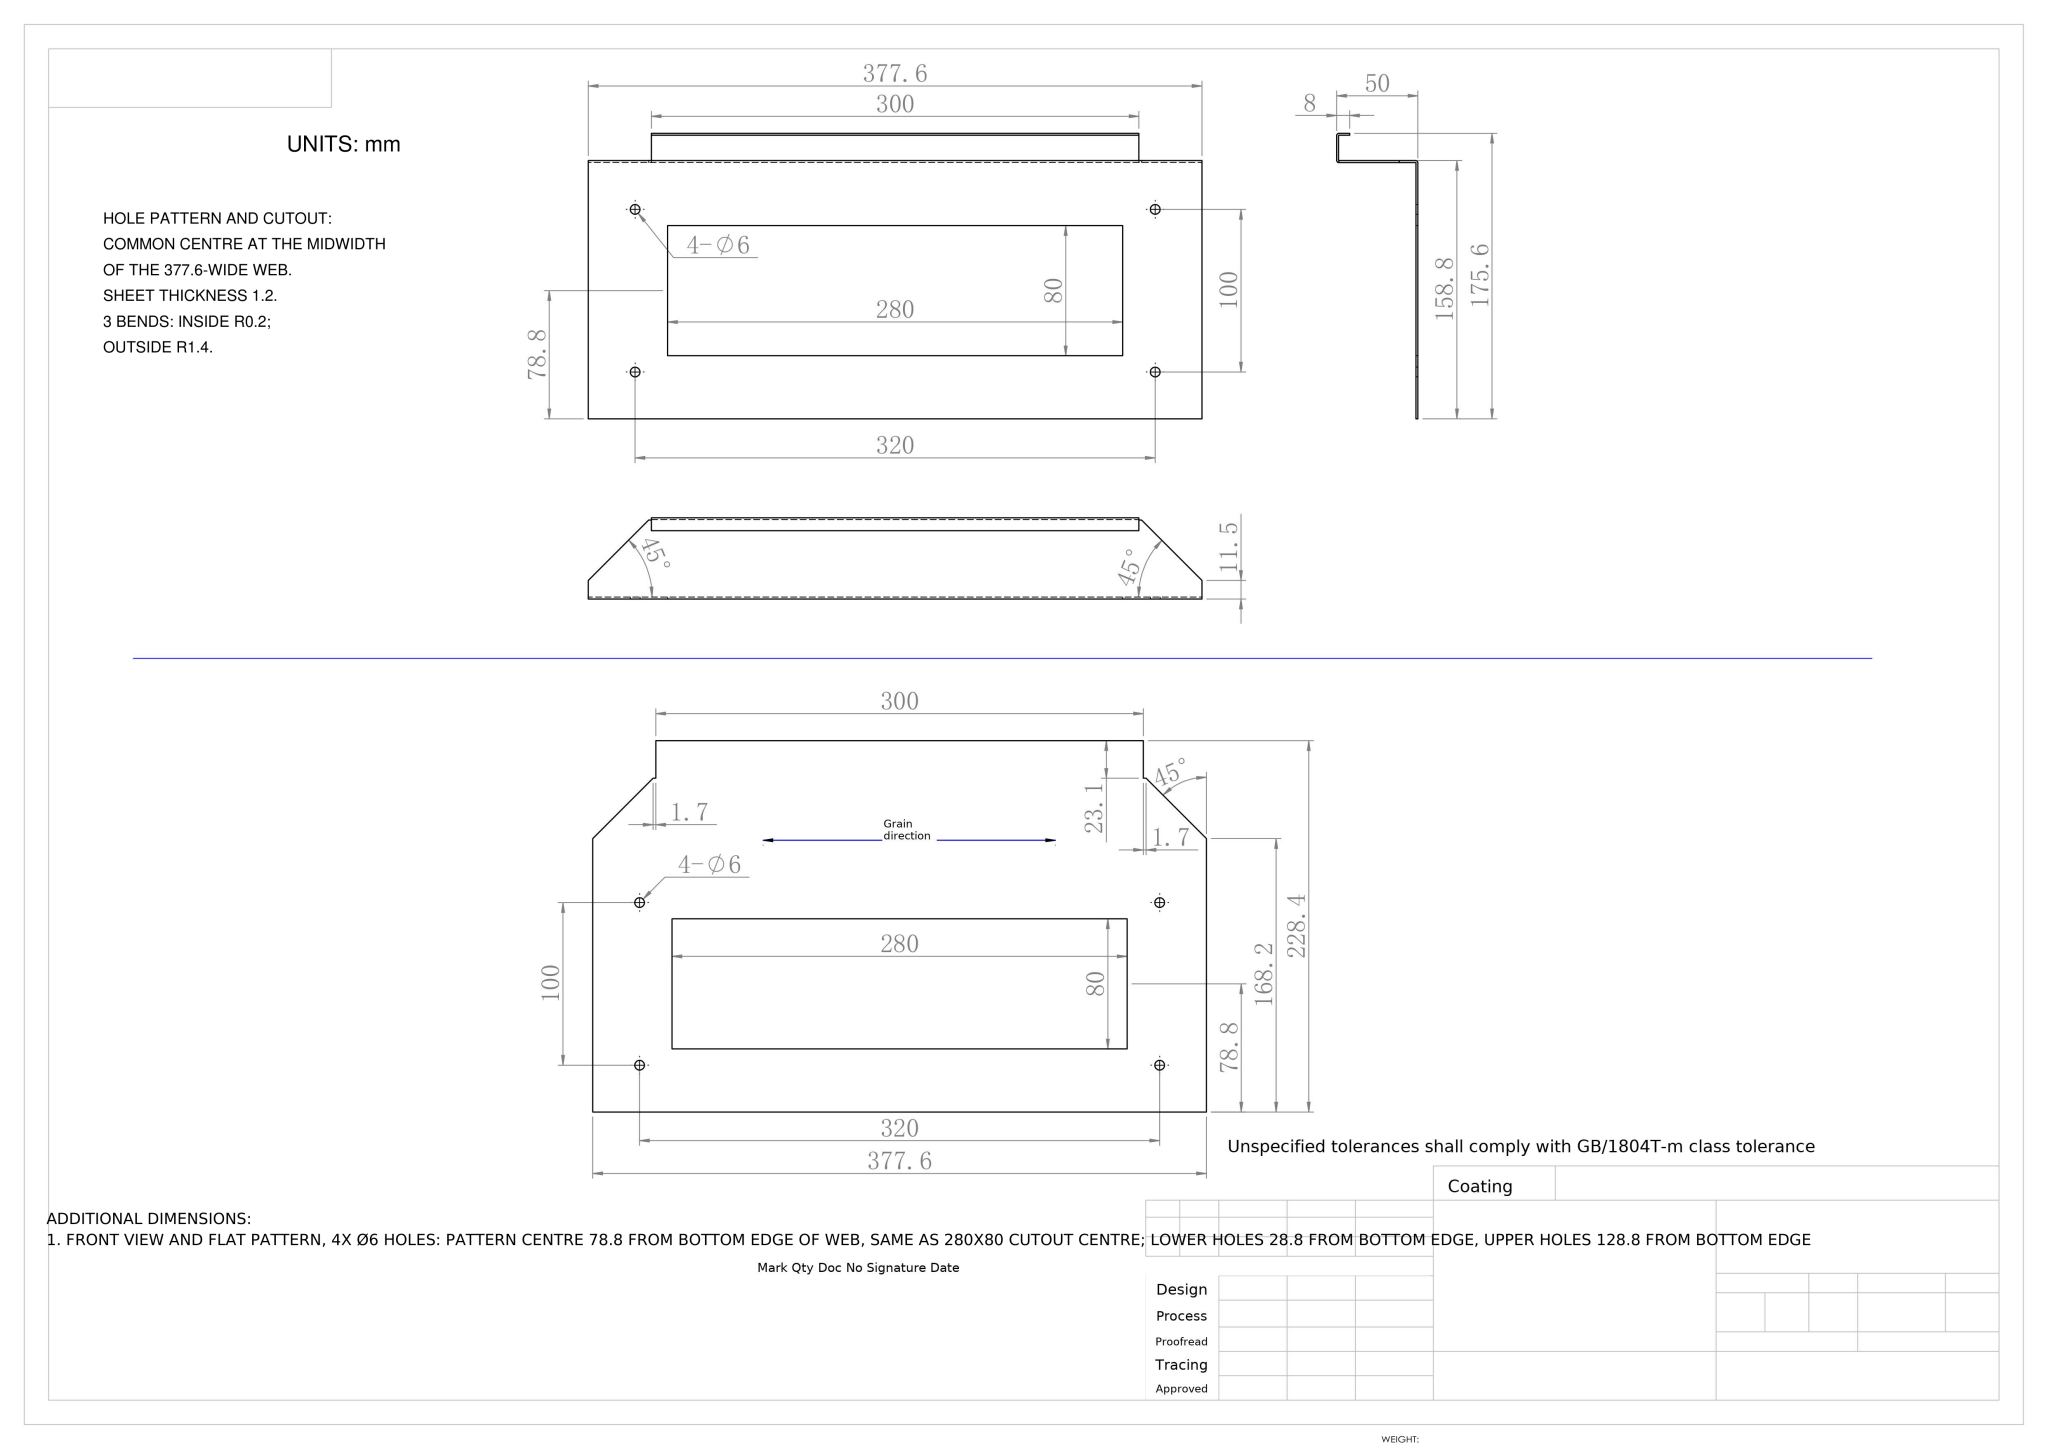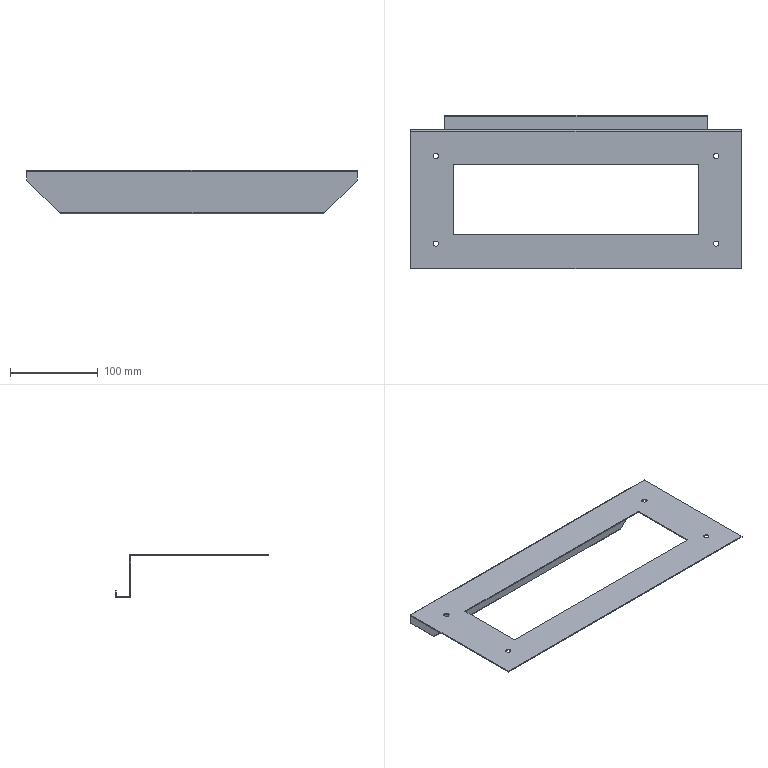Part | NX | mm | 1 solid | 46 faces | box 377.6 x 175.6 x 50 mm | volume 73363 mm3 | plane 32 | cylinder 14 | commonest cylinder face diameters 6 x8 2.8 x3 0.4 x3